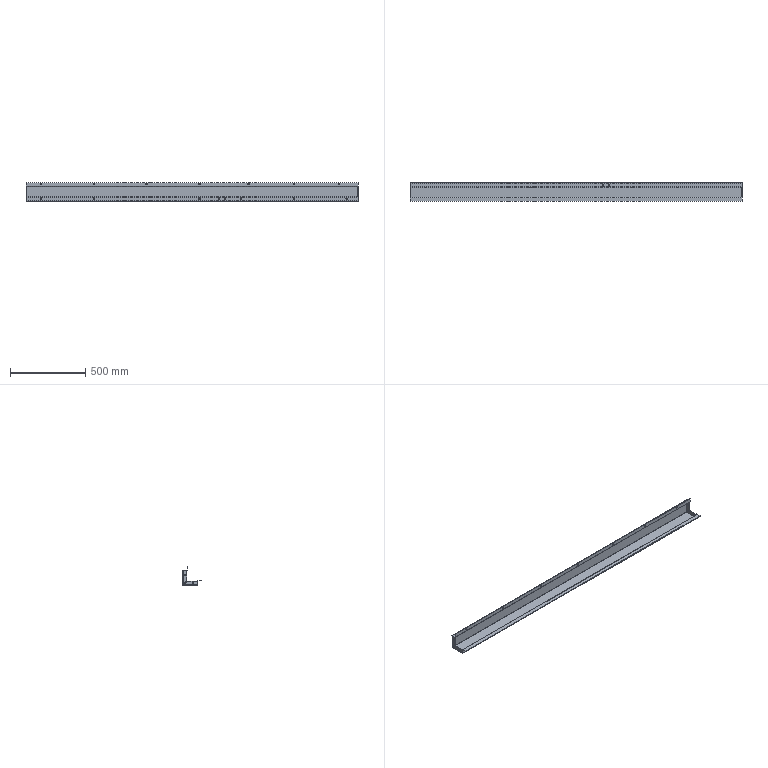Component | SolidWorks | 14RearUpperBeam-1 | 1 solid | 134 faces | volume 1349043 mm3 | cylinder 66 | plane 64 | spline 4 | commonest cylinder face diameters 10 x48 6 x9 2 x9